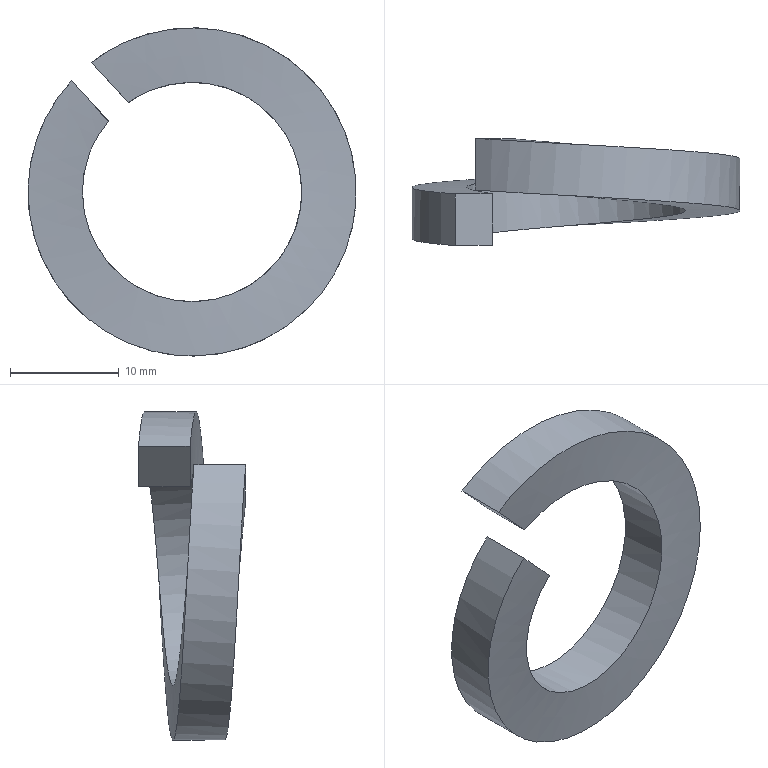Component | SolidWorks | GB_T93-1987StandardSpringWasher(Part)20_10-1 | 1 solid | 6 faces | box 30.21 x 9.87 x 30.21 mm | volume 1824 mm3 | spline 4 | plane 2
build123d program:
from build123d import *

# Parameters (mm, degrees)
BASE_EXTRUDE_DEPTH      = 0.001
BASE_EXTRUDE_DEPTH_BACK = 0.001
SKETCH6_W               = 4.71
SKETCH6_H               = 4.96
SWEEP3_PITCH            = 5.25
SWEEP3_HEIGHT           = 5.25
SWEEP3_RADIUS           = 10.1
SWEEP3_START_ANGLE      = 135
SKETCH7_W               = 4.75
SKETCH7_H               = 5
CUT_EXTRUDE1_DEPTH      = 22.997
CUT_EXTRUDE1_DEPTH_BACK = 22.997


with BuildPart() as part:
    # Sketch6 → Base-Extrude (new, two sides: drawn at the far end of the back side and taken through both)
    with BuildSketch(Plane(origin=(-7.142, 7.142, 5.25), x_dir=(0.0583, 0.0583, -0.9966), z_dir=(0.7047, 0.7047, 0.08245)).offset(-BASE_EXTRUDE_DEPTH_BACK)):
        with Locations((2.375, 2.5)):
            Rectangle(SKETCH6_W, SKETCH6_H)
    extrude(amount=BASE_EXTRUDE_DEPTH + BASE_EXTRUDE_DEPTH_BACK)

    # Sweep3: sweep along a helix
    with BuildLine() as sweep3_path:
        add(Helix(SWEEP3_PITCH, SWEEP3_HEIGHT, SWEEP3_RADIUS, center=(0, 0, 0), direction=(0, 0, 1), lefthand=True, mode=Mode.PRIVATE).rotate(Axis((0, 0, 0), (0, 0, 1)), SWEEP3_START_ANGLE))
    # Sketch7 → Sweep3 (sweep)
    with BuildSketch(Plane(origin=(-7.142, 7.142, 5.25), x_dir=(0.0583, 0.0583, -0.9966), z_dir=(0.7047, 0.7047, 0.08245))):
        with Locations((2.375, 2.5)):
            Rectangle(SKETCH7_W, SKETCH7_H)
    sweep(path=sweep3_path.line, is_frenet=True)

    # Sketch9 → Cut-Extrude1 (cut, two sides: drawn at the far end of the back side and taken through both)
    with BuildSketch(Plane.XY.offset(-CUT_EXTRUDE1_DEPTH_BACK)):
        Polygon((-34.367, 36.135), (0.6347, 1.133), (-1.133, -0.6347), (-37.903, 36.135), align=None)
    extrude(amount=CUT_EXTRUDE1_DEPTH + CUT_EXTRUDE1_DEPTH_BACK, mode=Mode.SUBTRACT)


solid = part.part

# Placed as in the assembly
solid = solid.moved(Location((-340.001, -183.818, 130.001), (90, -0.0006929, -2.365)))
STEP:
#1=CARTESIAN_POINT('',(-13.689,-7.44,5.375));
#2=VERTEX_POINT('',#1);
#3=CARTESIAN_POINT('',(-13.617,-7.241,5.442));
#4=VERTEX_POINT('',#3);
#5=CARTESIAN_POINT('',(-13.689,-7.44,5.375));
#6=CARTESIAN_POINT('',(-13.741,-7.433,5.314));
#7=CARTESIAN_POINT('',(-13.765,-7.426,5.237));
#8=CARTESIAN_POINT('',(-13.797,-7.418,5.135));
#9=CARTESIAN_POINT('',(-13.774,-7.409,5.031));
#10=CARTESIAN_POINT('',(-13.751,-7.401,4.927));
#11=CARTESIAN_POINT('',(-13.678,-7.392,4.849));
#12=CARTESIAN_POINT('',(-13.606,-7.383,4.77));
#13=CARTESIAN_POINT('',(-13.504,-7.375,4.739));
#14=CARTESIAN_POINT('',(-13.403,-7.366,4.707));
#15=CARTESIAN_POINT('',(-13.299,-7.358,4.73));
#16=CARTESIAN_POINT('',(-13.195,-7.349,4.753));
#17=CARTESIAN_POINT('',(-13.116,-7.34,4.826));
#18=CARTESIAN_POINT('',(-13.038,-7.332,4.898));
#19=CARTESIAN_POINT('',(-13.006,-7.323,4.999));
#20=CARTESIAN_POINT('',(-12.975,-7.314,5.101));
#21=CARTESIAN_POINT('',(-12.998,-7.306,5.205));
#22=CARTESIAN_POINT('',(-13.021,-7.297,5.309));
#23=CARTESIAN_POINT('',(-13.093,-7.289,5.387));
#24=CARTESIAN_POINT('',(-13.165,-7.28,5.466));
#25=CARTESIAN_POINT('',(-13.267,-7.271,5.498));
#26=CARTESIAN_POINT('',(-13.369,-7.263,5.529));
#27=CARTESIAN_POINT('',(-13.473,-7.254,5.506));
#28=CARTESIAN_POINT('',(-13.551,-7.248,5.489));
#29=CARTESIAN_POINT('',(-13.617,-7.241,5.442));
#30=(BOUNDED_CURVE()B_SPLINE_CURVE(2,(#5,#6,#7,#8,#9,#10,#11,#12,#13,#14,#15,#16,#17,#18,#19,#20,#21,#22,#23,#24,#25,#26,#27,#28,#29),.UNSPECIFIED.,.F.,.F.)B_SPLINE_CURVE_WITH_KNOTS((3,2,2,2,2,2,2,2,2,2,2,2,3),(0.01984,0.08333,0.1667,0.25,0.3333,0.4167,0.5,0.5833,0.6667,0.75,0.8333,0.9167,0.9802),.UNSPECIFIED.)CURVE()GEOMETRIC_REPRESENTATION_ITEM()RATIONAL_B_SPLINE_CURVE((0.9876,0.974,1.,0.9659,1.,0.9659,1.,0.9659,1.,0.9659,1.,0.9659,1.,0.9659,1.,0.9659,1.,0.9659,1.,0.9659,1.,0.9659,1.,0.974,0.9876))REPRESENTATION_ITEM(''));
#31=EDGE_CURVE('',#2,#4,#30,.T.);
#32=ORIENTED_EDGE('',*,*,#31,.F.);
#33=CARTESIAN_POINT('',(-13.823,-7.441,5.521));
#34=VERTEX_POINT('',#33);
#35=CARTESIAN_POINT('',(-13.689,-7.44,5.375));
#36=CARTESIAN_POINT('',(-13.701,-7.44,5.388));
#37=CARTESIAN_POINT('',(-13.712,-7.44,5.4));
#38=CARTESIAN_POINT('',(-13.724,-7.44,5.413));
#39=CARTESIAN_POINT('',(-13.735,-7.44,5.425));
#40=CARTESIAN_POINT('',(-13.747,-7.44,5.438));
#41=CARTESIAN_POINT('',(-13.758,-7.44,5.45));
#42=CARTESIAN_POINT('',(-13.78,-7.441,5.474));
#43=CARTESIAN_POINT('',(-13.802,-7.441,5.497));
#44=CARTESIAN_POINT('',(-13.823,-7.441,5.521));
#45=B_SPLINE_CURVE_WITH_KNOTS('',3,(#35,#36,#37,#38,#39,#40,#41,#42,#43,#44),.UNSPECIFIED.,.F.,.F.,(4,3,3,4),(0.,0.001294,0.002588,0.005026),.UNSPECIFIED.);
#46=EDGE_CURVE('',#2,#34,#45,.T.);
#47=ORIENTED_EDGE('',*,*,#46,.T.);
#48=CARTESIAN_POINT('',(-13.751,-7.24,5.587));
#49=VERTEX_POINT('',#48);
#50=CARTESIAN_POINT('',(-13.823,-7.441,5.521));
#51=CARTESIAN_POINT('',(-13.913,-7.434,5.423));
#52=CARTESIAN_POINT('',(-13.953,-7.426,5.296));
#53=CARTESIAN_POINT('',(-14.001,-7.418,5.143));
#54=CARTESIAN_POINT('',(-13.966,-7.409,4.988));
#55=CARTESIAN_POINT('',(-13.931,-7.401,4.833));
#56=CARTESIAN_POINT('',(-13.823,-7.392,4.715));
#57=CARTESIAN_POINT('',(-13.715,-7.383,4.598));
#58=CARTESIAN_POINT('',(-13.563,-7.375,4.551));
#59=CARTESIAN_POINT('',(-13.411,-7.366,4.503));
#60=CARTESIAN_POINT('',(-13.256,-7.358,4.538));
#61=CARTESIAN_POINT('',(-13.1,-7.349,4.573));
#62=CARTESIAN_POINT('',(-12.983,-7.34,4.681));
#63=CARTESIAN_POINT('',(-12.866,-7.332,4.789));
#64=CARTESIAN_POINT('',(-12.818,-7.323,4.941));
#65=CARTESIAN_POINT('',(-12.771,-7.314,5.093));
#66=CARTESIAN_POINT('',(-12.806,-7.306,5.248));
#67=CARTESIAN_POINT('',(-12.841,-7.297,5.404));
#68=CARTESIAN_POINT('',(-12.948,-7.289,5.521));
#69=CARTESIAN_POINT('',(-13.056,-7.28,5.638));
#70=CARTESIAN_POINT('',(-13.208,-7.271,5.686));
#71=CARTESIAN_POINT('',(-13.36,-7.263,5.733));
#72=CARTESIAN_POINT('',(-13.516,-7.254,5.698));
#73=CARTESIAN_POINT('',(-13.646,-7.247,5.669));
#74=CARTESIAN_POINT('',(-13.751,-7.24,5.587));
#75=(BOUNDED_CURVE()B_SPLINE_CURVE(2,(#50,#51,#52,#53,#54,#55,#56,#57,#58,#59,#60,#61,#62,#63,#64,#65,#66,#67,#68,#69,#70,#71,#72,#73,#74),.UNSPECIFIED.,.F.,.F.)B_SPLINE_CURVE_WITH_KNOTS((3,2,2,2,2,2,2,2,2,2,2,2,3),(0.01328,0.08333,0.1667,0.25,0.3333,0.4167,0.5,0.5833,0.6667,0.75,0.8333,0.9167,0.9867),.UNSPECIFIED.)CURVE()GEOMETRIC_REPRESENTATION_ITEM()RATIONAL_B_SPLINE_CURVE((0.9909,0.9714,1.,0.9659,1.,0.9659,1.,0.9659,1.,0.9659,1.,0.9659,1.,0.9659,1.,0.9659,1.,0.9659,1.,0.9659,1.,0.9659,1.,0.9714,0.9909))REPRESENTATION_ITEM(''));
#76=EDGE_CURVE('',#34,#49,#75,.T.);
#77=ORIENTED_EDGE('',*,*,#76,.T.);
#78=CARTESIAN_POINT('',(-13.751,-7.24,5.587));
#79=CARTESIAN_POINT('',(-13.739,-7.24,5.575));
#80=CARTESIAN_POINT('',(-13.728,-7.24,5.562));
#81=CARTESIAN_POINT('',(-13.716,-7.24,5.55));
#82=CARTESIAN_POINT('',(-13.705,-7.24,5.537));
#83=CARTESIAN_POINT('',(-13.693,-7.24,5.525));
#84=CARTESIAN_POINT('',(-13.682,-7.24,5.512));
#85=CARTESIAN_POINT('',(-13.66,-7.24,5.489));
#86=CARTESIAN_POINT('',(-13.639,-7.241,5.465));
#87=CARTESIAN_POINT('',(-13.617,-7.241,5.442));
#88=B_SPLINE_CURVE_WITH_KNOTS('',3,(#78,#79,#80,#81,#82,#83,#84,#85,#86,#87),.UNSPECIFIED.,.F.,.F.,(4,3,3,4),(0.,0.001294,0.002588,0.005026),.UNSPECIFIED.);
#89=EDGE_CURVE('',#49,#4,#88,.T.);
#90=ORIENTED_EDGE('',*,*,#89,.T.);
#91=EDGE_LOOP('',(#32,#47,#77,#90));
#92=FACE_OUTER_BOUND('',#91,.T.);
#93=CARTESIAN_POINT('',(-13.789,-7.444,5.555));
#94=CARTESIAN_POINT('',(-13.906,-7.435,5.448));
#95=CARTESIAN_POINT('',(-13.953,-7.426,5.296));
#96=CARTESIAN_POINT('',(-14.001,-7.418,5.143));
#97=CARTESIAN_POINT('',(-13.966,-7.409,4.988));
#98=CARTESIAN_POINT('',(-13.931,-7.401,4.833));
#99=CARTESIAN_POINT('',(-13.823,-7.392,4.715));
#100=CARTESIAN_POINT('',(-13.715,-7.383,4.598));
#101=CARTESIAN_POINT('',(-13.563,-7.375,4.551));
#102=CARTESIAN_POINT('',(-13.411,-7.366,4.503));
#103=CARTESIAN_POINT('',(-13.256,-7.358,4.538));
#104=CARTESIAN_POINT('',(-13.1,-7.349,4.573));
#105=CARTESIAN_POINT('',(-12.983,-7.34,4.681));
#106=CARTESIAN_POINT('',(-12.866,-7.332,4.789));
#107=CARTESIAN_POINT('',(-12.818,-7.323,4.941));
#108=CARTESIAN_POINT('',(-12.771,-7.314,5.093));
#109=CARTESIAN_POINT('',(-12.806,-7.306,5.248));
#110=CARTESIAN_POINT('',(-12.841,-7.297,5.404));
#111=CARTESIAN_POINT('',(-12.948,-7.289,5.521));
#112=CARTESIAN_POINT('',(-13.056,-7.28,5.638));
#113=CARTESIAN_POINT('',(-13.208,-7.271,5.686));
#114=CARTESIAN_POINT('',(-13.36,-7.263,5.733));
#115=CARTESIAN_POINT('',(-13.516,-7.254,5.698));
#116=CARTESIAN_POINT('',(-13.671,-7.246,5.663));
#117=CARTESIAN_POINT('',(-13.789,-7.237,5.555));
#118=CARTESIAN_POINT('',(-13.655,-7.444,5.411));
#119=CARTESIAN_POINT('',(-13.734,-7.435,5.338));
#120=CARTESIAN_POINT('',(-13.765,-7.426,5.237));
#121=CARTESIAN_POINT('',(-13.797,-7.418,5.135));
#122=CARTESIAN_POINT('',(-13.774,-7.409,5.031));
#123=CARTESIAN_POINT('',(-13.751,-7.401,4.927));
#124=CARTESIAN_POINT('',(-13.678,-7.392,4.849));
#125=CARTESIAN_POINT('',(-13.606,-7.383,4.77));
#126=CARTESIAN_POINT('',(-13.504,-7.375,4.739));
#127=CARTESIAN_POINT('',(-13.403,-7.366,4.707));
#128=CARTESIAN_POINT('',(-13.299,-7.358,4.73));
#129=CARTESIAN_POINT('',(-13.195,-7.349,4.753));
#130=CARTESIAN_POINT('',(-13.116,-7.34,4.826));
#131=CARTESIAN_POINT('',(-13.038,-7.332,4.898));
#132=CARTESIAN_POINT('',(-13.006,-7.323,4.999));
#133=CARTESIAN_POINT('',(-12.975,-7.314,5.101));
#134=CARTESIAN_POINT('',(-12.998,-7.306,5.205));
#135=CARTESIAN_POINT('',(-13.021,-7.297,5.309));
#136=CARTESIAN_POINT('',(-13.093,-7.289,5.387));
#137=CARTESIAN_POINT('',(-13.165,-7.28,5.466));
#138=CARTESIAN_POINT('',(-13.267,-7.271,5.498));
#139=CARTESIAN_POINT('',(-13.369,-7.263,5.529));
#140=CARTESIAN_POINT('',(-13.473,-7.254,5.506));
#141=CARTESIAN_POINT('',(-13.577,-7.246,5.483));
#142=CARTESIAN_POINT('',(-13.655,-7.237,5.411));
#143=(BOUNDED_SURFACE()B_SPLINE_SURFACE(1,2,((#93,#94,#95,#96,#97,#98,#99,#100,#101,#102,#103,#104,#105,#106,#107,#108,#109,#110,#111,#112,#113,#114,#115,#116,#117),(#118,#119,#120,#121,#122,#123,#124,#125,#126,#127,#128,#129,#130,#131,#132,#133,#134,#135,#136,#137,#138,#139,#140,#141,#142)),.UNSPECIFIED.,.F.,.F.,.F.)B_SPLINE_SURFACE_WITH_KNOTS((2,2),(3,2,2,2,2,2,2,2,2,2,2,2,3),(0.,0.2564),(0.,0.08333,0.1667,0.25,0.3333,0.4167,0.5,0.5833,0.6667,0.75,0.8333,0.9167,1.),.UNSPECIFIED.)GEOMETRIC_REPRESENTATION_ITEM()RATIONAL_B_SPLINE_SURFACE(((1.,0.9659,1.,0.9659,1.,0.9659,1.,0.9659,1.,0.9659,1.,0.9659,1.,0.9659,1.,0.9659,1.,0.9659,1.,0.9659,1.,0.9659,1.,0.9659,1.),(1.,0.9659,1.,0.9659,1.,0.9659,1.,0.9659,1.,0.9659,1.,0.9659,1.,0.9659,1.,0.9659,1.,0.9659,1.,0.9659,1.,0.9659,1.,0.9659,1.)))REPRESENTATION_ITEM('')SURFACE());
#144=ADVANCED_FACE('',(#92),#143,.F.);
#145=CARTESIAN_POINT('',(-13.69,-7.252,5.375));
#146=VERTEX_POINT('',#145);
#147=CARTESIAN_POINT('',(-13.617,-7.053,5.442));
#148=VERTEX_POINT('',#147);
#149=CARTESIAN_POINT('',(-13.69,-7.252,5.375));
#150=CARTESIAN_POINT('',(-13.736,-7.246,5.32));
#151=CARTESIAN_POINT('',(-13.761,-7.24,5.251));
#152=CARTESIAN_POINT('',(-13.796,-7.231,5.151));
#153=CARTESIAN_POINT('',(-13.777,-7.223,5.046));
#154=CARTESIAN_POINT('',(-13.758,-7.214,4.941));
#155=CARTESIAN_POINT('',(-13.689,-7.206,4.86));
#156=CARTESIAN_POINT('',(-13.62,-7.197,4.779));
#157=CARTESIAN_POINT('',(-13.519,-7.188,4.743));
#158=CARTESIAN_POINT('',(-13.419,-7.18,4.707));
#159=CARTESIAN_POINT('',(-13.314,-7.171,4.727));
#160=CARTESIAN_POINT('',(-13.209,-7.163,4.746));
#161=CARTESIAN_POINT('',(-13.128,-7.154,4.815));
#162=CARTESIAN_POINT('',(-13.047,-7.145,4.884));
#163=CARTESIAN_POINT('',(-13.011,-7.137,4.985));
#164=CARTESIAN_POINT('',(-12.975,-7.128,5.085));
#165=CARTESIAN_POINT('',(-12.994,-7.119,5.19));
#166=CARTESIAN_POINT('',(-13.014,-7.111,5.295));
#167=CARTESIAN_POINT('',(-13.083,-7.102,5.376));
#168=CARTESIAN_POINT('',(-13.152,-7.094,5.457));
#169=CARTESIAN_POINT('',(-13.252,-7.085,5.493));
#170=CARTESIAN_POINT('',(-13.353,-7.076,5.529));
#171=CARTESIAN_POINT('',(-13.458,-7.068,5.509));
#172=CARTESIAN_POINT('',(-13.545,-7.061,5.493));
#173=CARTESIAN_POINT('',(-13.617,-7.053,5.442));
#174=(BOUNDED_CURVE()B_SPLINE_CURVE(2,(#149,#150,#151,#152,#153,#154,#155,#156,#157,#158,#159,#160,#161,#162,#163,#164,#165,#166,#167,#168,#169,#170,#171,#172,#173),.UNSPECIFIED.,.F.,.T.)B_SPLINE_CURVE_WITH_KNOTS((3,2,2,2,2,2,2,2,2,2,2,2,3),(0.02598,0.08333,0.1667,0.25,0.3333,0.4167,0.5,0.5833,0.6667,0.75,0.8333,0.9167,0.9863),.UNSPECIFIED.)CURVE()GEOMETRIC_REPRESENTATION_ITEM()RATIONAL_B_SPLINE_CURVE((0.9854,0.9765,1.,0.9659,1.,0.9659,1.,0.9659,1.,0.9659,1.,0.9659,1.,0.9659,1.,0.9659,1.,0.9659,1.,0.9659,1.,0.9659,1.,0.9715,0.9907))REPRESENTATION_ITEM(''));
#175=EDGE_CURVE('',#146,#148,#174,.T.);
#176=ORIENTED_EDGE('',*,*,#175,.F.);
#177=CARTESIAN_POINT('',(-13.69,-7.252,5.375));
#178=CARTESIAN_POINT('',(-13.689,-7.268,5.375));
#179=CARTESIAN_POINT('',(-13.689,-7.283,5.375));
#180=CARTESIAN_POINT('',(-13.689,-7.299,5.375));
#181=CARTESIAN_POINT('',(-13.689,-7.322,5.375));
#182=CARTESIAN_POINT('',(-13.689,-7.346,5.375));
#183=CARTESIAN_POINT('',(-13.689,-7.369,5.375));
#184=CARTESIAN_POINT('',(-13.689,-7.393,5.375));
#185=CARTESIAN_POINT('',(-13.689,-7.416,5.375));
#186=CARTESIAN_POINT('',(-13.689,-7.44,5.375));
#187=B_SPLINE_CURVE_WITH_KNOTS('',3,(#177,#178,#179,#180,#181,#182,#183,#184,#185,#186),.UNSPECIFIED.,.F.,.F.,(4,3,3,4),(0.,0.001192,0.002979,0.004766),.UNSPECIFIED.);
#188=EDGE_CURVE('',#146,#2,#187,.T.);
#189=ORIENTED_EDGE('',*,*,#188,.T.);
#190=ORIENTED_EDGE('',*,*,#31,.T.);
#191=CARTESIAN_POINT('',(-13.617,-7.241,5.442));
#192=CARTESIAN_POINT('',(-13.617,-7.21,5.442));
#193=CARTESIAN_POINT('',(-13.617,-7.178,5.442));
#194=CARTESIAN_POINT('',(-13.617,-7.147,5.442));
#195=CARTESIAN_POINT('',(-13.617,-7.132,5.442));
#196=CARTESIAN_POINT('',(-13.617,-7.116,5.442));
#197=CARTESIAN_POINT('',(-13.617,-7.1,5.442));
#198=CARTESIAN_POINT('',(-13.617,-7.085,5.442));
#199=CARTESIAN_POINT('',(-13.617,-7.069,5.442));
#200=CARTESIAN_POINT('',(-13.617,-7.053,5.442));
#201=B_SPLINE_CURVE_WITH_KNOTS('',3,(#191,#192,#193,#194,#195,#196,#197,#198,#199,#200),.UNSPECIFIED.,.F.,.F.,(4,3,3,4),(0.,0.002383,0.003575,0.004766),.UNSPECIFIED.);
#202=EDGE_CURVE('',#4,#148,#201,.T.);
#203=ORIENTED_EDGE('',*,*,#202,.T.);
#204=EDGE_LOOP('',(#176,#189,#190,#203));
#205=FACE_OUTER_BOUND('',#204,.T.);
#206=CARTESIAN_POINT('',(-13.655,-7.444,5.411));
#207=CARTESIAN_POINT('',(-13.734,-7.435,5.338));
#208=CARTESIAN_POINT('',(-13.765,-7.426,5.237));
#209=CARTESIAN_POINT('',(-13.797,-7.418,5.135));
#210=CARTESIAN_POINT('',(-13.774,-7.409,5.031));
#211=CARTESIAN_POINT('',(-13.751,-7.401,4.927));
#212=CARTESIAN_POINT('',(-13.678,-7.392,4.849));
#213=CARTESIAN_POINT('',(-13.606,-7.383,4.77));
#214=CARTESIAN_POINT('',(-13.504,-7.375,4.739));
#215=CARTESIAN_POINT('',(-13.403,-7.366,4.707));
#216=CARTESIAN_POINT('',(-13.299,-7.358,4.73));
#217=CARTESIAN_POINT('',(-13.195,-7.349,4.753));
#218=CARTESIAN_POINT('',(-13.116,-7.34,4.826));
#219=CARTESIAN_POINT('',(-13.038,-7.332,4.898));
#220=CARTESIAN_POINT('',(-13.006,-7.323,4.999));
#221=CARTESIAN_POINT('',(-12.975,-7.314,5.101));
#222=CARTESIAN_POINT('',(-12.998,-7.306,5.205));
#223=CARTESIAN_POINT('',(-13.021,-7.297,5.309));
#224=CARTESIAN_POINT('',(-13.093,-7.289,5.387));
#225=CARTESIAN_POINT('',(-13.165,-7.28,5.466));
#226=CARTESIAN_POINT('',(-13.267,-7.271,5.498));
#227=CARTESIAN_POINT('',(-13.369,-7.263,5.529));
#228=CARTESIAN_POINT('',(-13.473,-7.254,5.506));
#229=CARTESIAN_POINT('',(-13.577,-7.246,5.483));
#230=CARTESIAN_POINT('',(-13.655,-7.237,5.411));
#231=CARTESIAN_POINT('',(-13.644,-7.257,5.421));
#232=CARTESIAN_POINT('',(-13.725,-7.249,5.352));
#233=CARTESIAN_POINT('',(-13.761,-7.24,5.251));
#234=CARTESIAN_POINT('',(-13.796,-7.231,5.151));
#235=CARTESIAN_POINT('',(-13.777,-7.223,5.046));
#236=CARTESIAN_POINT('',(-13.758,-7.214,4.941));
#237=CARTESIAN_POINT('',(-13.689,-7.206,4.86));
#238=CARTESIAN_POINT('',(-13.62,-7.197,4.779));
#239=CARTESIAN_POINT('',(-13.519,-7.188,4.743));
#240=CARTESIAN_POINT('',(-13.419,-7.18,4.707));
#241=CARTESIAN_POINT('',(-13.314,-7.171,4.727));
#242=CARTESIAN_POINT('',(-13.209,-7.163,4.746));
#243=CARTESIAN_POINT('',(-13.128,-7.154,4.815));
#244=CARTESIAN_POINT('',(-13.047,-7.145,4.884));
#245=CARTESIAN_POINT('',(-13.011,-7.137,4.985));
#246=CARTESIAN_POINT('',(-12.975,-7.128,5.085));
#247=CARTESIAN_POINT('',(-12.994,-7.119,5.19));
#248=CARTESIAN_POINT('',(-13.014,-7.111,5.295));
#249=CARTESIAN_POINT('',(-13.083,-7.102,5.376));
#250=CARTESIAN_POINT('',(-13.152,-7.094,5.457));
#251=CARTESIAN_POINT('',(-13.252,-7.085,5.493));
#252=CARTESIAN_POINT('',(-13.353,-7.076,5.529));
#253=CARTESIAN_POINT('',(-13.458,-7.068,5.509));
#254=CARTESIAN_POINT('',(-13.563,-7.059,5.49));
#255=CARTESIAN_POINT('',(-13.644,-7.051,5.421));
#256=(BOUNDED_SURFACE()B_SPLINE_SURFACE(1,2,((#206,#207,#208,#209,#210,#211,#212,#213,#214,#215,#216,#217,#218,#219,#220,#221,#222,#223,#224,#225,#226,#227,#228,#229,#230),(#231,#232,#233,#234,#235,#236,#237,#238,#239,#240,#241,#242,#243,#244,#245,#246,#247,#248,#249,#250,#251,#252,#253,#254,#255)),.UNSPECIFIED.,.F.,.F.,.F.)B_SPLINE_SURFACE_WITH_KNOTS((2,2),(3,2,2,2,2,2,2,2,2,2,2,2,3),(0.2564,0.5),(0.,0.08333,0.1667,0.25,0.3333,0.4167,0.5,0.5833,0.6667,0.75,0.8333,0.9167,1.),.UNSPECIFIED.)GEOMETRIC_REPRESENTATION_ITEM()RATIONAL_B_SPLINE_SURFACE(((1.,0.9659,1.,0.9659,1.,0.9659,1.,0.9659,1.,0.9659,1.,0.9659,1.,0.9659,1.,0.9659,1.,0.9659,1.,0.9659,1.,0.9659,1.,0.9659,1.),(1.,0.9659,1.,0.9659,1.,0.9659,1.,0.9659,1.,0.9659,1.,0.9659,1.,0.9659,1.,0.9659,1.,0.9659,1.,0.9659,1.,0.9659,1.,0.9659,1.)))REPRESENTATION_ITEM('')SURFACE());
#257=ADVANCED_FACE('',(#205),#256,.F.);
#258=CARTESIAN_POINT('',(-13.823,-7.254,5.521));
#259=VERTEX_POINT('',#258);
#260=CARTESIAN_POINT('',(-13.751,-7.052,5.587));
#261=VERTEX_POINT('',#260);
#262=CARTESIAN_POINT('',(-13.823,-7.254,5.521));
#263=CARTESIAN_POINT('',(-13.908,-7.247,5.429));
#264=CARTESIAN_POINT('',(-13.949,-7.24,5.31));
#265=CARTESIAN_POINT('',(-14.,-7.231,5.159));
#266=CARTESIAN_POINT('',(-13.969,-7.223,5.003));
#267=CARTESIAN_POINT('',(-13.938,-7.214,4.847));
#268=CARTESIAN_POINT('',(-13.834,-7.206,4.727));
#269=CARTESIAN_POINT('',(-13.729,-7.197,4.607));
#270=CARTESIAN_POINT('',(-13.578,-7.188,4.555));
#271=CARTESIAN_POINT('',(-13.427,-7.18,4.504));
#272=CARTESIAN_POINT('',(-13.271,-7.171,4.535));
#273=CARTESIAN_POINT('',(-13.114,-7.163,4.565));
#274=CARTESIAN_POINT('',(-12.994,-7.154,4.67));
#275=CARTESIAN_POINT('',(-12.875,-7.145,4.775));
#276=CARTESIAN_POINT('',(-12.823,-7.137,4.926));
#277=CARTESIAN_POINT('',(-12.772,-7.128,5.077));
#278=CARTESIAN_POINT('',(-12.802,-7.119,5.233));
#279=CARTESIAN_POINT('',(-12.833,-7.111,5.389));
#280=CARTESIAN_POINT('',(-12.938,-7.102,5.509));
#281=CARTESIAN_POINT('',(-13.043,-7.094,5.629));
#282=CARTESIAN_POINT('',(-13.194,-7.085,5.681));
#283=CARTESIAN_POINT('',(-13.345,-7.076,5.732));
#284=CARTESIAN_POINT('',(-13.501,-7.068,5.702));
#285=CARTESIAN_POINT('',(-13.64,-7.06,5.674));
#286=CARTESIAN_POINT('',(-13.751,-7.052,5.587));
#287=(BOUNDED_CURVE()B_SPLINE_CURVE(2,(#262,#263,#264,#265,#266,#267,#268,#269,#270,#271,#272,#273,#274,#275,#276,#277,#278,#279,#280,#281,#282,#283,#284,#285,#286),.UNSPECIFIED.,.F.,.T.)B_SPLINE_CURVE_WITH_KNOTS((3,2,2,2,2,2,2,2,2,2,2,2,3),(0.0174,0.08333,0.1667,0.25,0.3333,0.4167,0.5,0.5833,0.6667,0.75,0.8333,0.9167,0.9909),.UNSPECIFIED.)CURVE()GEOMETRIC_REPRESENTATION_ITEM()RATIONAL_B_SPLINE_CURVE((0.9887,0.973,1.,0.9659,1.,0.9659,1.,0.9659,1.,0.9659,1.,0.9659,1.,0.9659,1.,0.9659,1.,0.9659,1.,0.9659,1.,0.9659,1.,0.9697,0.9934))REPRESENTATION_ITEM(''));
#288=EDGE_CURVE('',#259,#261,#287,.T.);
#289=ORIENTED_EDGE('',*,*,#288,.F.);
#290=CARTESIAN_POINT('',(-13.823,-7.254,5.521));
#291=CARTESIAN_POINT('',(-13.812,-7.254,5.508));
#292=CARTESIAN_POINT('',(-13.8,-7.254,5.496));
#293=CARTESIAN_POINT('',(-13.789,-7.253,5.483));
#294=CARTESIAN_POINT('',(-13.777,-7.253,5.471));
#295=CARTESIAN_POINT('',(-13.766,-7.253,5.458));
#296=CARTESIAN_POINT('',(-13.754,-7.253,5.446));
#297=CARTESIAN_POINT('',(-13.733,-7.253,5.422));
#298=CARTESIAN_POINT('',(-13.711,-7.252,5.399));
#299=CARTESIAN_POINT('',(-13.69,-7.252,5.375));
#300=B_SPLINE_CURVE_WITH_KNOTS('',3,(#290,#291,#292,#293,#294,#295,#296,#297,#298,#299),.UNSPECIFIED.,.F.,.F.,(4,3,3,4),(0.,0.001294,0.002588,0.005023),.UNSPECIFIED.);
#301=EDGE_CURVE('',#259,#146,#300,.T.);
#302=ORIENTED_EDGE('',*,*,#301,.T.);
#303=ORIENTED_EDGE('',*,*,#175,.T.);
#304=CARTESIAN_POINT('',(-13.617,-7.053,5.442));
#305=CARTESIAN_POINT('',(-13.629,-7.053,5.454));
#306=CARTESIAN_POINT('',(-13.64,-7.053,5.467));
#307=CARTESIAN_POINT('',(-13.652,-7.053,5.479));
#308=CARTESIAN_POINT('',(-13.663,-7.053,5.492));
#309=CARTESIAN_POINT('',(-13.675,-7.053,5.504));
#310=CARTESIAN_POINT('',(-13.686,-7.053,5.517));
#311=CARTESIAN_POINT('',(-13.708,-7.053,5.54));
#312=CARTESIAN_POINT('',(-13.729,-7.053,5.564));
#313=CARTESIAN_POINT('',(-13.751,-7.052,5.587));
#314=B_SPLINE_CURVE_WITH_KNOTS('',3,(#304,#305,#306,#307,#308,#309,#310,#311,#312,#313),.UNSPECIFIED.,.F.,.F.,(4,3,3,4),(0.,0.001294,0.002588,0.005023),.UNSPECIFIED.);
#315=EDGE_CURVE('',#148,#261,#314,.T.);
#316=ORIENTED_EDGE('',*,*,#315,.T.);
#317=EDGE_LOOP('',(#289,#302,#303,#316));
#318=FACE_OUTER_BOUND('',#317,.T.);
#319=CARTESIAN_POINT('',(-13.644,-7.257,5.421));
#320=CARTESIAN_POINT('',(-13.725,-7.249,5.352));
#321=CARTESIAN_POINT('',(-13.761,-7.24,5.251));
#322=CARTESIAN_POINT('',(-13.796,-7.231,5.151));
#323=CARTESIAN_POINT('',(-13.777,-7.223,5.046));
#324=CARTESIAN_POINT('',(-13.758,-7.214,4.941));
#325=CARTESIAN_POINT('',(-13.689,-7.206,4.86));
#326=CARTESIAN_POINT('',(-13.62,-7.197,4.779));
#327=CARTESIAN_POINT('',(-13.519,-7.188,4.743));
#328=CARTESIAN_POINT('',(-13.419,-7.18,4.707));
#329=CARTESIAN_POINT('',(-13.314,-7.171,4.727));
#330=CARTESIAN_POINT('',(-13.209,-7.163,4.746));
#331=CARTESIAN_POINT('',(-13.128,-7.154,4.815));
#332=CARTESIAN_POINT('',(-13.047,-7.145,4.884));
#333=CARTESIAN_POINT('',(-13.011,-7.137,4.985));
#334=CARTESIAN_POINT('',(-12.975,-7.128,5.085));
#335=CARTESIAN_POINT('',(-12.994,-7.119,5.19));
#336=CARTESIAN_POINT('',(-13.014,-7.111,5.295));
#337=CARTESIAN_POINT('',(-13.083,-7.102,5.376));
#338=CARTESIAN_POINT('',(-13.152,-7.094,5.457));
#339=CARTESIAN_POINT('',(-13.252,-7.085,5.493));
#340=CARTESIAN_POINT('',(-13.353,-7.076,5.529));
#341=CARTESIAN_POINT('',(-13.458,-7.068,5.509));
#342=CARTESIAN_POINT('',(-13.563,-7.059,5.49));
#343=CARTESIAN_POINT('',(-13.644,-7.051,5.421));
#344=CARTESIAN_POINT('',(-13.777,-7.257,5.566));
#345=CARTESIAN_POINT('',(-13.897,-7.249,5.461));
#346=CARTESIAN_POINT('',(-13.949,-7.24,5.31));
#347=CARTESIAN_POINT('',(-14.,-7.231,5.159));
#348=CARTESIAN_POINT('',(-13.969,-7.223,5.003));
#349=CARTESIAN_POINT('',(-13.938,-7.214,4.847));
#350=CARTESIAN_POINT('',(-13.834,-7.206,4.727));
#351=CARTESIAN_POINT('',(-13.729,-7.197,4.607));
#352=CARTESIAN_POINT('',(-13.578,-7.188,4.555));
#353=CARTESIAN_POINT('',(-13.427,-7.18,4.504));
#354=CARTESIAN_POINT('',(-13.271,-7.171,4.535));
#355=CARTESIAN_POINT('',(-13.114,-7.163,4.565));
#356=CARTESIAN_POINT('',(-12.994,-7.154,4.67));
#357=CARTESIAN_POINT('',(-12.875,-7.145,4.775));
#358=CARTESIAN_POINT('',(-12.823,-7.137,4.926));
#359=CARTESIAN_POINT('',(-12.772,-7.128,5.077));
#360=CARTESIAN_POINT('',(-12.802,-7.119,5.233));
#361=CARTESIAN_POINT('',(-12.833,-7.111,5.389));
#362=CARTESIAN_POINT('',(-12.938,-7.102,5.509));
#363=CARTESIAN_POINT('',(-13.043,-7.094,5.629));
#364=CARTESIAN_POINT('',(-13.194,-7.085,5.681));
#365=CARTESIAN_POINT('',(-13.345,-7.076,5.732));
#366=CARTESIAN_POINT('',(-13.501,-7.068,5.702));
#367=CARTESIAN_POINT('',(-13.657,-7.059,5.671));
#368=CARTESIAN_POINT('',(-13.777,-7.051,5.566));
#369=(BOUNDED_SURFACE()B_SPLINE_SURFACE(1,2,((#319,#320,#321,#322,#323,#324,#325,#326,#327,#328,#329,#330,#331,#332,#333,#334,#335,#336,#337,#338,#339,#340,#341,#342,#343),(#344,#345,#346,#347,#348,#349,#350,#351,#352,#353,#354,#355,#356,#357,#358,#359,#360,#361,#362,#363,#364,#365,#366,#367,#368)),.UNSPECIFIED.,.F.,.F.,.T.)B_SPLINE_SURFACE_WITH_KNOTS((2,2),(3,2,2,2,2,2,2,2,2,2,2,2,3),(0.5,0.7564),(0.,0.08333,0.1667,0.25,0.3333,0.4167,0.5,0.5833,0.6667,0.75,0.8333,0.9167,1.),.UNSPECIFIED.)GEOMETRIC_REPRESENTATION_ITEM()RATIONAL_B_SPLINE_SURFACE(((1.,0.9659,1.,0.9659,1.,0.9659,1.,0.9659,1.,0.9659,1.,0.9659,1.,0.9659,1.,0.9659,1.,0.9659,1.,0.9659,1.,0.9659,1.,0.9659,1.),(1.,0.9659,1.,0.9659,1.,0.9659,1.,0.9659,1.,0.9659,1.,0.9659,1.,0.9659,1.,0.9659,1.,0.9659,1.,0.9659,1.,0.9659,1.,0.9659,1.)))REPRESENTATION_ITEM('')SURFACE());
#370=ADVANCED_FACE('',(#318),#369,.F.);
#371=ORIENTED_EDGE('',*,*,#76,.F.);
#372=CARTESIAN_POINT('',(-13.823,-7.441,5.521));
#373=CARTESIAN_POINT('',(-13.823,-7.425,5.521));
#374=CARTESIAN_POINT('',(-13.823,-7.41,5.521));
#375=CARTESIAN_POINT('',(-13.823,-7.394,5.521));
#376=CARTESIAN_POINT('',(-13.823,-7.371,5.521));
#377=CARTESIAN_POINT('',(-13.823,-7.347,5.521));
#378=CARTESIAN_POINT('',(-13.823,-7.324,5.521));
#379=CARTESIAN_POINT('',(-13.823,-7.301,5.521));
#380=CARTESIAN_POINT('',(-13.823,-7.277,5.521));
#381=CARTESIAN_POINT('',(-13.823,-7.254,5.521));
#382=B_SPLINE_CURVE_WITH_KNOTS('',3,(#372,#373,#374,#375,#376,#377,#378,#379,#380,#381),.UNSPECIFIED.,.F.,.F.,(4,3,3,4),(0.,0.001189,0.002972,0.004755),.UNSPECIFIED.);
#383=EDGE_CURVE('',#34,#259,#382,.T.);
#384=ORIENTED_EDGE('',*,*,#383,.T.);
#385=ORIENTED_EDGE('',*,*,#288,.T.);
#386=CARTESIAN_POINT('',(-13.751,-7.052,5.587));
#387=CARTESIAN_POINT('',(-13.751,-7.068,5.587));
#388=CARTESIAN_POINT('',(-13.751,-7.084,5.587));
#389=CARTESIAN_POINT('',(-13.751,-7.099,5.587));
#390=CARTESIAN_POINT('',(-13.751,-7.123,5.587));
#391=CARTESIAN_POINT('',(-13.751,-7.146,5.587));
#392=CARTESIAN_POINT('',(-13.751,-7.169,5.587));
#393=CARTESIAN_POINT('',(-13.751,-7.193,5.587));
#394=CARTESIAN_POINT('',(-13.751,-7.216,5.587));
#395=CARTESIAN_POINT('',(-13.751,-7.24,5.587));
#396=B_SPLINE_CURVE_WITH_KNOTS('',3,(#386,#387,#388,#389,#390,#391,#392,#393,#394,#395),.UNSPECIFIED.,.F.,.F.,(4,3,3,4),(0.,0.001189,0.002972,0.004755),.UNSPECIFIED.);
#397=EDGE_CURVE('',#261,#49,#396,.T.);
#398=ORIENTED_EDGE('',*,*,#397,.T.);
#399=EDGE_LOOP('',(#371,#384,#385,#398));
#400=FACE_OUTER_BOUND('',#399,.T.);
#401=CARTESIAN_POINT('',(-13.777,-7.257,5.566));
#402=CARTESIAN_POINT('',(-13.897,-7.249,5.461));
#403=CARTESIAN_POINT('',(-13.949,-7.24,5.31));
#404=CARTESIAN_POINT('',(-14.,-7.231,5.159));
#405=CARTESIAN_POINT('',(-13.969,-7.223,5.003));
#406=CARTESIAN_POINT('',(-13.938,-7.214,4.847));
#407=CARTESIAN_POINT('',(-13.834,-7.206,4.727));
#408=CARTESIAN_POINT('',(-13.729,-7.197,4.607));
#409=CARTESIAN_POINT('',(-13.578,-7.188,4.555));
#410=CARTESIAN_POINT('',(-13.427,-7.18,4.504));
#411=CARTESIAN_POINT('',(-13.271,-7.171,4.535));
#412=CARTESIAN_POINT('',(-13.114,-7.163,4.565));
#413=CARTESIAN_POINT('',(-12.994,-7.154,4.67));
#414=CARTESIAN_POINT('',(-12.875,-7.145,4.775));
#415=CARTESIAN_POINT('',(-12.823,-7.137,4.926));
#416=CARTESIAN_POINT('',(-12.772,-7.128,5.077));
#417=CARTESIAN_POINT('',(-12.802,-7.119,5.233));
#418=CARTESIAN_POINT('',(-12.833,-7.111,5.389));
#419=CARTESIAN_POINT('',(-12.938,-7.102,5.509));
#420=CARTESIAN_POINT('',(-13.043,-7.094,5.629));
#421=CARTESIAN_POINT('',(-13.194,-7.085,5.681));
#422=CARTESIAN_POINT('',(-13.345,-7.076,5.732));
#423=CARTESIAN_POINT('',(-13.501,-7.068,5.702));
#424=CARTESIAN_POINT('',(-13.657,-7.059,5.671));
#425=CARTESIAN_POINT('',(-13.777,-7.051,5.566));
#426=CARTESIAN_POINT('',(-13.789,-7.444,5.555));
#427=CARTESIAN_POINT('',(-13.906,-7.435,5.448));
#428=CARTESIAN_POINT('',(-13.953,-7.426,5.296));
#429=CARTESIAN_POINT('',(-14.001,-7.418,5.143));
#430=CARTESIAN_POINT('',(-13.966,-7.409,4.988));
#431=CARTESIAN_POINT('',(-13.931,-7.401,4.833));
#432=CARTESIAN_POINT('',(-13.823,-7.392,4.715));
#433=CARTESIAN_POINT('',(-13.715,-7.383,4.598));
#434=CARTESIAN_POINT('',(-13.563,-7.375,4.551));
#435=CARTESIAN_POINT('',(-13.411,-7.366,4.503));
#436=CARTESIAN_POINT('',(-13.256,-7.358,4.538));
#437=CARTESIAN_POINT('',(-13.1,-7.349,4.573));
#438=CARTESIAN_POINT('',(-12.983,-7.34,4.681));
#439=CARTESIAN_POINT('',(-12.866,-7.332,4.789));
#440=CARTESIAN_POINT('',(-12.818,-7.323,4.941));
#441=CARTESIAN_POINT('',(-12.771,-7.314,5.093));
#442=CARTESIAN_POINT('',(-12.806,-7.306,5.248));
#443=CARTESIAN_POINT('',(-12.841,-7.297,5.404));
#444=CARTESIAN_POINT('',(-12.948,-7.289,5.521));
#445=CARTESIAN_POINT('',(-13.056,-7.28,5.638));
#446=CARTESIAN_POINT('',(-13.208,-7.271,5.686));
#447=CARTESIAN_POINT('',(-13.36,-7.263,5.733));
#448=CARTESIAN_POINT('',(-13.516,-7.254,5.698));
#449=CARTESIAN_POINT('',(-13.671,-7.246,5.663));
#450=CARTESIAN_POINT('',(-13.789,-7.237,5.555));
#451=(BOUNDED_SURFACE()B_SPLINE_SURFACE(1,2,((#401,#402,#403,#404,#405,#406,#407,#408,#409,#410,#411,#412,#413,#414,#415,#416,#417,#418,#419,#420,#421,#422,#423,#424,#425),(#426,#427,#428,#429,#430,#431,#432,#433,#434,#435,#436,#437,#438,#439,#440,#441,#442,#443,#444,#445,#446,#447,#448,#449,#450)),.UNSPECIFIED.,.F.,.F.,.F.)B_SPLINE_SURFACE_WITH_KNOTS((2,2),(3,2,2,2,2,2,2,2,2,2,2,2,3),(0.7564,1.),(0.,0.08333,0.1667,0.25,0.3333,0.4167,0.5,0.5833,0.6667,0.75,0.8333,0.9167,1.),.UNSPECIFIED.)GEOMETRIC_REPRESENTATION_ITEM()RATIONAL_B_SPLINE_SURFACE(((1.,0.9659,1.,0.9659,1.,0.9659,1.,0.9659,1.,0.9659,1.,0.9659,1.,0.9659,1.,0.9659,1.,0.9659,1.,0.9659,1.,0.9659,1.,0.9659,1.),(1.,0.9659,1.,0.9659,1.,0.9659,1.,0.9659,1.,0.9659,1.,0.9659,1.,0.9659,1.,0.9659,1.,0.9659,1.,0.9659,1.,0.9659,1.,0.9659,1.)))REPRESENTATION_ITEM('')SURFACE());
#452=ADVANCED_FACE('',(#400),#451,.F.);
#453=ORIENTED_EDGE('',*,*,#397,.F.);
#454=ORIENTED_EDGE('',*,*,#315,.F.);
#455=ORIENTED_EDGE('',*,*,#202,.F.);
#456=ORIENTED_EDGE('',*,*,#89,.F.);
#457=EDGE_LOOP('',(#453,#454,#455,#456));
#458=FACE_OUTER_BOUND('',#457,.T.);
#459=CARTESIAN_POINT('',(-14.679,-7.05,6.595));
#460=DIRECTION('',(0.7357,0.,0.6774));
#461=DIRECTION('',(-0.6774,-0.,0.7357));
#462=AXIS2_PLACEMENT_3D('',#459,#460,#461);
#463=PLANE('',#462);
#464=ADVANCED_FACE('',(#458),#463,.F.);
#465=ORIENTED_EDGE('',*,*,#188,.F.);
#466=ORIENTED_EDGE('',*,*,#301,.F.);
#467=ORIENTED_EDGE('',*,*,#383,.F.);
#468=ORIENTED_EDGE('',*,*,#46,.F.);
#469=EDGE_LOOP('',(#465,#466,#467,#468));
#470=FACE_OUTER_BOUND('',#469,.T.);
#471=CARTESIAN_POINT('',(-13.431,-7.05,5.095));
#472=DIRECTION('',(-0.7357,-0.,-0.6774));
#473=DIRECTION('',(0.6774,0.,-0.7357));
#474=AXIS2_PLACEMENT_3D('',#471,#472,#473);
#475=PLANE('',#474);
#476=ADVANCED_FACE('',(#470),#475,.F.);
#477=CLOSED_SHELL('',(#144,#257,#370,#452,#464,#476));
#478=MANIFOLD_SOLID_BREP('',#477);
#479=CARTESIAN_POINT('',(0.,0.,0.));
#480=DIRECTION('',(0.,0.,1.));
#481=DIRECTION('',(1.,0.,0.));
#482=AXIS2_PLACEMENT_3D('',#479,#480,#481);
#483=(LENGTH_UNIT()NAMED_UNIT(*)SI_UNIT($,.METRE.));
#484=LENGTH_MEASURE_WITH_UNIT(LENGTH_MEASURE(0.0254),#483);
#485=DIMENSIONAL_EXPONENTS(1.,0.,0.,0.,0.,0.,0.);
#486=(CONVERSION_BASED_UNIT('',#484)LENGTH_UNIT()NAMED_UNIT(#485));
#487=UNCERTAINTY_MEASURE_WITH_UNIT(LENGTH_MEASURE(0.00001),#486,'','');
#488=(NAMED_UNIT(*)PLANE_ANGLE_UNIT()SI_UNIT($,.RADIAN.));
#489=(NAMED_UNIT(*)SI_UNIT($,.STERADIAN.)SOLID_ANGLE_UNIT());
#490=(GEOMETRIC_REPRESENTATION_CONTEXT(3)GLOBAL_UNCERTAINTY_ASSIGNED_CONTEXT((#487))GLOBAL_UNIT_ASSIGNED_CONTEXT((#486,#488,#489))REPRESENTATION_CONTEXT('',''));
#491=ADVANCED_BREP_SHAPE_REPRESENTATION('',(#478,#482),#490);
#492=COLOUR_RGB('',0.7922,0.8196,0.9333);
#493=FILL_AREA_STYLE_COLOUR('',#492);
#494=FILL_AREA_STYLE('',(#493));
#495=SURFACE_STYLE_FILL_AREA(#494);
#496=SURFACE_SIDE_STYLE('',(#495));
#497=SURFACE_STYLE_USAGE(.BOTH.,#496);
#498=PRESENTATION_STYLE_ASSIGNMENT((#497));
#499=STYLED_ITEM('',(#498),#478);
#500=PRESENTATION_LAYER_ASSIGNMENT('','',(#499));
#501=(LENGTH_UNIT()NAMED_UNIT(*)SI_UNIT($,.METRE.));
#502=LENGTH_MEASURE_WITH_UNIT(LENGTH_MEASURE(0.0254),#501);
#503=DIMENSIONAL_EXPONENTS(1.,0.,0.,0.,0.,0.,0.);
#504=(CONVERSION_BASED_UNIT('',#502)LENGTH_UNIT()NAMED_UNIT(#503));
#505=UNCERTAINTY_MEASURE_WITH_UNIT(LENGTH_MEASURE(0.00001),#504,'','');
#506=(NAMED_UNIT(*)PLANE_ANGLE_UNIT()SI_UNIT($,.RADIAN.));
#507=(NAMED_UNIT(*)SI_UNIT($,.STERADIAN.)SOLID_ANGLE_UNIT());
#508=(GEOMETRIC_REPRESENTATION_CONTEXT(3)GLOBAL_UNCERTAINTY_ASSIGNED_CONTEXT((#505))GLOBAL_UNIT_ASSIGNED_CONTEXT((#504,#506,#507))REPRESENTATION_CONTEXT('',''));
#509=MECHANICAL_DESIGN_GEOMETRIC_PRESENTATION_REPRESENTATION('',(#499),#508);